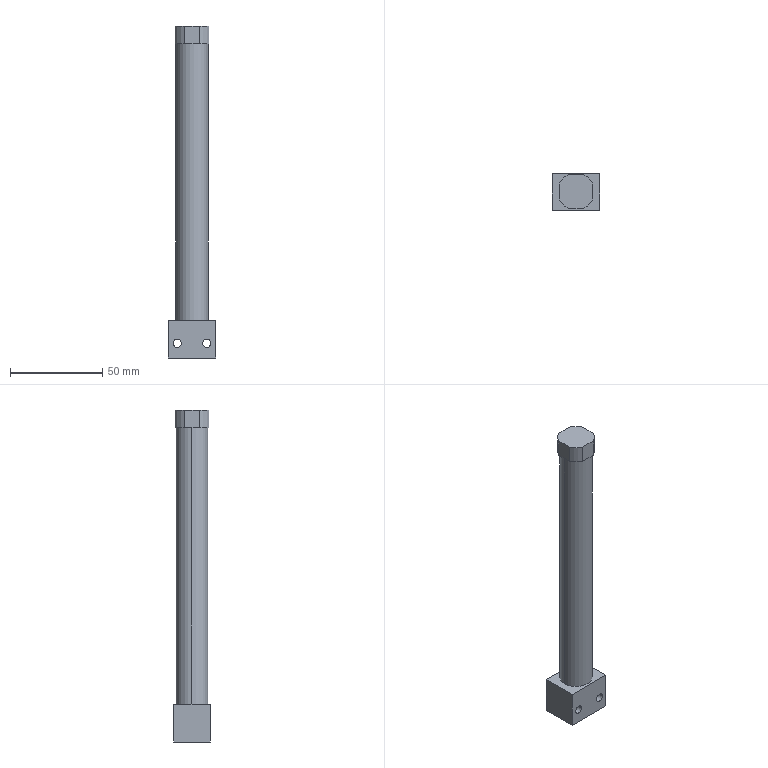Component | SolidWorks | F-YBCDJ2RKA16-125-M9NL(0_0_0)-1_F-YBCJ2RKA16-125-M9N(0_0)_BODY-1 | 1 solid | 46 faces | box 26 x 20 x 180 mm | volume 21278 mm3 | cylinder 22 | plane 16 | cone 8 | commonest cylinder face diameters 4.134 x4 8 x4 4.5 x4 20 x4 16 x2 6.004 x2 17.4 x2
build123d program:
from build123d import *

# Parameters (mm, degrees)
SKETCH1_W           = 26
SKETCH1_H           = 20
BOSS_EXTRUDE1_DEPTH = 20.5
HOLE1_D             = 4.5
HOLE1_CBORE_D       = 8
HOLE1_CBORE_DEPTH   = 5
HOLE2_D             = 4.5
HOLE2_CBORE_D       = 8
HOLE2_CBORE_DEPTH   = 5
SKETCH6_R           = 8.7
BOSS_EXTRUDE2_DEPTH = 150
BOSS_EXTRUDE3_DEPTH = 9.5
HOLE3_D             = 4.134
HOLE3_DEPTH         = 5.5
HOLE3_CSINK_D       = 5
HOLE3_CSINK_ANGLE   = 90
HOLE3_TIP           = 1.193
HOLE4_D             = 4.134
HOLE4_DEPTH         = 5.5
HOLE4_CSINK_D       = 5
HOLE4_CSINK_ANGLE   = 90
HOLE4_TIP           = 1.193


with BuildPart() as part:
    # Sketch1 → Boss-Extrude1 (new body)
    with BuildSketch(Plane(origin=(0, 0, 0), x_dir=(0, 0, -1), z_dir=(1, 0, 0))):
        Rectangle(SKETCH1_W, SKETCH1_H)
    extrude(amount=BOSS_EXTRUDE1_DEPTH)

    # Hole1 (through all)
    with Locations(Plane(origin=(0, 10, 0), x_dir=(1, 0, 0), z_dir=(0, 1, 0))):
        with Locations((8, 8)):
            CounterBoreHole(HOLE1_D / 2, HOLE1_CBORE_D / 2, HOLE1_CBORE_DEPTH)

    # Hole2 (through all)
    with Locations(Plane(origin=(0, 10, 0), x_dir=(1, 0, 0), z_dir=(0, 1, 0))):
        with Locations((8, -8)):
            CounterBoreHole(HOLE2_D / 2, HOLE2_CBORE_D / 2, HOLE2_CBORE_DEPTH)

    # Sketch6 → Boss-Extrude2 (add)
    with BuildSketch(Plane(origin=(20.5, 0, 0), x_dir=(0, 0, -1), z_dir=(1, 0, 0))):
        Circle(SKETCH6_R)
    extrude(amount=BOSS_EXTRUDE2_DEPTH)

    # Sketch7 → Boss-Extrude3 (add)
    with BuildSketch(Plane(origin=(170.5, 0, 0), x_dir=(0, 0, -1), z_dir=(1, 0, 0))):
        with BuildLine():
            Line((-4.035, -9.15), (4.035, -9.15))
            ThreePointArc((4.035, -9.15), (7.071, -7.071), (9.15, -4.035))
            Line((9.15, -4.035), (9.15, 4.035))
            ThreePointArc((9.15, 4.035), (7.071, 7.071), (4.035, 9.15))
            Line((4.035, 9.15), (-4.035, 9.15))
            ThreePointArc((-4.035, 9.15), (-7.071, 7.071), (-9.15, 4.035))
            Line((-9.15, 4.035), (-9.15, -4.035))
            ThreePointArc((-9.15, -4.035), (-7.071, -7.071), (-4.035, -9.15))
        make_face()
    extrude(amount=BOSS_EXTRUDE3_DEPTH)

    # Hole3
    with Locations(Plane(origin=(0, 10, 0), x_dir=(1, 0, 0), z_dir=(0, 1, 0))):
        with Locations((16, 0)):
            CounterSinkHole(HOLE3_D / 2, HOLE3_CSINK_D / 2, depth=HOLE3_DEPTH, counter_sink_angle=HOLE3_CSINK_ANGLE)
            with Locations((0, 0, -(HOLE3_DEPTH + HOLE3_TIP / 2))):  # 120° drill point
                Cone(0, HOLE3_D / 2, HOLE3_TIP, mode=Mode.SUBTRACT)

    # Hole4
    with Locations(Plane(origin=(0, 9.15, 0), x_dir=(1, 0, 0), z_dir=(0, 1, 0))):
        with Locations((175, 0)):
            CounterSinkHole(HOLE4_D / 2, HOLE4_CSINK_D / 2, depth=HOLE4_DEPTH, counter_sink_angle=HOLE4_CSINK_ANGLE)
            with Locations((0, 0, -(HOLE4_DEPTH + HOLE4_TIP / 2))):  # 120° drill point
                Cone(0, HOLE4_D / 2, HOLE4_TIP, mode=Mode.SUBTRACT)

    # Sketch12 → Cut-Revolve1 (revolve, cut)
    with BuildSketch(Plane.XY, mode=Mode.PRIVATE) as cut_revolve1_sk:
        Polygon((0, 0), (0, 3.002), (20.5, 3.002), (20.5, 8), (150.5, 8), (150.5, 0), align=None)
    revolve(cut_revolve1_sk.sketch.rotate(Axis((50, 0, 0), (-1, 0, 0)), 270), axis=Axis((50, 0, 0), (-1, 0, 0)), mode=Mode.SUBTRACT)


solid = part.part

# Placed as in the assembly
solid = solid.moved(Location((272.305, 302.175, 226.479), (0, -90, 0)))